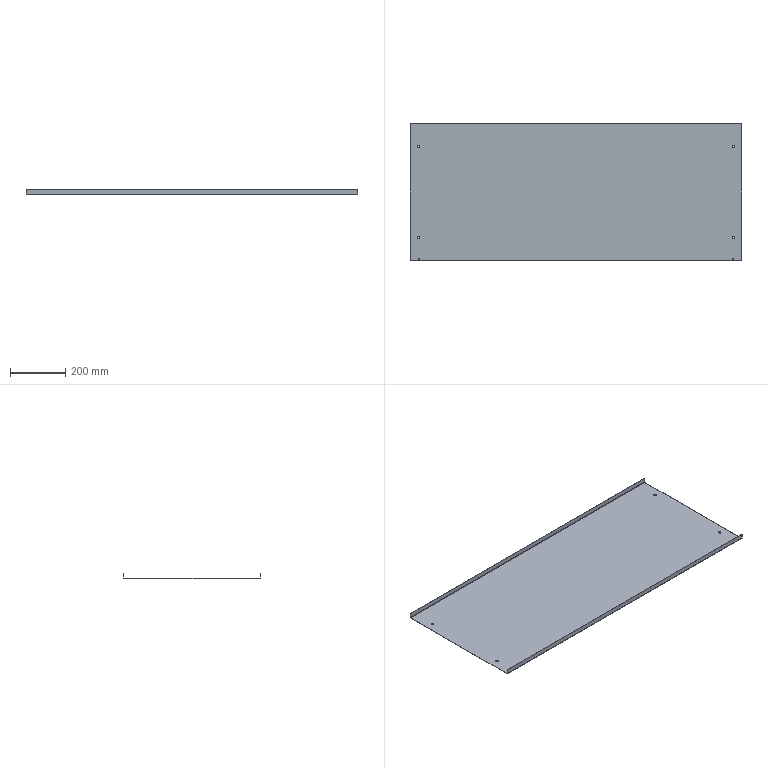Component | SolidWorks | TopPlate-1_TopPanelInnerPanel-2_TopPanelInnerPanel-1 | 1 solid | 34 faces | box 1198 x 498 x 18.5 mm | volume 509853 mm3 | plane 18 | cylinder 16 | commonest cylinder face diameters 8 x8 6 x4 2 x2 3.6 x2 | material 304
STEP:
#1=COLOUR_RGB('',0.7922,0.8196,0.9333);
#2=FILL_AREA_STYLE_COLOUR('',#1);
#3=FILL_AREA_STYLE('',(#2));
#4=SURFACE_STYLE_FILL_AREA(#3);
#5=SURFACE_SIDE_STYLE('',(#4));
#6=SURFACE_STYLE_USAGE(.BOTH.,#5);
#7=PRESENTATION_STYLE_ASSIGNMENT((#6));
#8=CARTESIAN_POINT('',(19.958,-8.263,78.498));
#9=VERTEX_POINT('',#8);
#10=CARTESIAN_POINT('',(19.958,-8.027,78.498));
#11=VERTEX_POINT('',#10);
#12=CARTESIAN_POINT('',(19.958,-8.145,78.498));
#13=DIRECTION('',(-0.,-0.,1.));
#14=DIRECTION('',(0.,1.,0.));
#15=AXIS2_PLACEMENT_3D('',#12,#13,#14);
#16=CIRCLE('',#15,0.1181);
#17=EDGE_CURVE('',#9,#11,#16,.T.);
#18=ORIENTED_EDGE('',*,*,#17,.T.);
#19=CARTESIAN_POINT('',(19.958,-8.027,78.467));
#20=VERTEX_POINT('',#19);
#21=CARTESIAN_POINT('',(19.958,-8.027,78.86));
#22=DIRECTION('',(0.,0.,-1.));
#23=VECTOR('',#22,39.37);
#24=LINE('',#21,#23);
#25=EDGE_CURVE('',#11,#20,#24,.T.);
#26=ORIENTED_EDGE('',*,*,#25,.T.);
#27=CARTESIAN_POINT('',(19.958,-8.263,78.467));
#28=VERTEX_POINT('',#27);
#29=CARTESIAN_POINT('',(19.958,-8.145,78.467));
#30=DIRECTION('',(0.,0.,-1.));
#31=DIRECTION('',(0.,-1.,0.));
#32=AXIS2_PLACEMENT_3D('',#29,#30,#31);
#33=CIRCLE('',#32,0.1181);
#34=EDGE_CURVE('',#20,#28,#33,.T.);
#35=ORIENTED_EDGE('',*,*,#34,.T.);
#36=CARTESIAN_POINT('',(19.958,-8.263,78.86));
#37=DIRECTION('',(0.,0.,-1.));
#38=VECTOR('',#37,39.37);
#39=LINE('',#36,#38);
#40=EDGE_CURVE('',#9,#28,#39,.T.);
#41=ORIENTED_EDGE('',*,*,#40,.F.);
#42=EDGE_LOOP('',(#18,#26,#35,#41));
#43=FACE_OUTER_BOUND('',#42,.T.);
#44=CARTESIAN_POINT('',(19.958,-8.145,78.86));
#45=DIRECTION('',(0.,0.,-1.));
#46=DIRECTION('',(0.,-1.,0.));
#47=AXIS2_PLACEMENT_3D('',#44,#45,#46);
#48=CYLINDRICAL_SURFACE('',#47,0.1181);
#49=ADVANCED_FACE('',(#43),#48,.F.);
#50=CARTESIAN_POINT('',(-24.688,-8.263,78.498));
#51=VERTEX_POINT('',#50);
#52=CARTESIAN_POINT('',(-24.688,-8.027,78.498));
#53=VERTEX_POINT('',#52);
#54=CARTESIAN_POINT('',(-24.688,-8.145,78.498));
#55=DIRECTION('',(-0.,-0.,1.));
#56=DIRECTION('',(0.,1.,0.));
#57=AXIS2_PLACEMENT_3D('',#54,#55,#56);
#58=CIRCLE('',#57,0.1181);
#59=EDGE_CURVE('',#51,#53,#58,.T.);
#60=ORIENTED_EDGE('',*,*,#59,.T.);
#61=CARTESIAN_POINT('',(-24.688,-8.027,78.467));
#62=VERTEX_POINT('',#61);
#63=CARTESIAN_POINT('',(-24.688,-8.027,78.86));
#64=DIRECTION('',(0.,0.,-1.));
#65=VECTOR('',#64,39.37);
#66=LINE('',#63,#65);
#67=EDGE_CURVE('',#53,#62,#66,.T.);
#68=ORIENTED_EDGE('',*,*,#67,.T.);
#69=CARTESIAN_POINT('',(-24.688,-8.263,78.467));
#70=VERTEX_POINT('',#69);
#71=CARTESIAN_POINT('',(-24.688,-8.145,78.467));
#72=DIRECTION('',(0.,0.,-1.));
#73=DIRECTION('',(0.,-1.,0.));
#74=AXIS2_PLACEMENT_3D('',#71,#72,#73);
#75=CIRCLE('',#74,0.1181);
#76=EDGE_CURVE('',#62,#70,#75,.T.);
#77=ORIENTED_EDGE('',*,*,#76,.T.);
#78=CARTESIAN_POINT('',(-24.688,-8.263,78.86));
#79=DIRECTION('',(0.,0.,-1.));
#80=VECTOR('',#79,39.37);
#81=LINE('',#78,#80);
#82=EDGE_CURVE('',#51,#70,#81,.T.);
#83=ORIENTED_EDGE('',*,*,#82,.F.);
#84=EDGE_LOOP('',(#60,#68,#77,#83));
#85=FACE_OUTER_BOUND('',#84,.T.);
#86=CARTESIAN_POINT('',(-24.688,-8.145,78.86));
#87=DIRECTION('',(0.,0.,-1.));
#88=DIRECTION('',(0.,-1.,0.));
#89=AXIS2_PLACEMENT_3D('',#86,#87,#88);
#90=CYLINDRICAL_SURFACE('',#89,0.1181);
#91=ADVANCED_FACE('',(#85),#90,.F.);
#92=CARTESIAN_POINT('',(-24.766,-5.29,78.498));
#93=VERTEX_POINT('',#92);
#94=CARTESIAN_POINT('',(-24.766,-4.975,78.498));
#95=VERTEX_POINT('',#94);
#96=CARTESIAN_POINT('',(-24.766,-5.133,78.498));
#97=DIRECTION('',(-0.,-0.,1.));
#98=DIRECTION('',(0.,1.,0.));
#99=AXIS2_PLACEMENT_3D('',#96,#97,#98);
#100=CIRCLE('',#99,0.1575);
#101=EDGE_CURVE('',#93,#95,#100,.T.);
#102=ORIENTED_EDGE('',*,*,#101,.T.);
#103=CARTESIAN_POINT('',(-24.766,-4.975,78.467));
#104=VERTEX_POINT('',#103);
#105=CARTESIAN_POINT('',(-24.766,-4.975,78.86));
#106=DIRECTION('',(0.,0.,-1.));
#107=VECTOR('',#106,39.37);
#108=LINE('',#105,#107);
#109=EDGE_CURVE('',#95,#104,#108,.T.);
#110=ORIENTED_EDGE('',*,*,#109,.T.);
#111=CARTESIAN_POINT('',(-24.766,-5.29,78.467));
#112=VERTEX_POINT('',#111);
#113=CARTESIAN_POINT('',(-24.766,-5.133,78.467));
#114=DIRECTION('',(0.,0.,-1.));
#115=DIRECTION('',(0.,1.,0.));
#116=AXIS2_PLACEMENT_3D('',#113,#114,#115);
#117=CIRCLE('',#116,0.1575);
#118=EDGE_CURVE('',#104,#112,#117,.T.);
#119=ORIENTED_EDGE('',*,*,#118,.T.);
#120=CARTESIAN_POINT('',(-24.766,-5.29,78.86));
#121=DIRECTION('',(0.,0.,-1.));
#122=VECTOR('',#121,39.37);
#123=LINE('',#120,#122);
#124=EDGE_CURVE('',#93,#112,#123,.T.);
#125=ORIENTED_EDGE('',*,*,#124,.F.);
#126=EDGE_LOOP('',(#102,#110,#119,#125));
#127=FACE_OUTER_BOUND('',#126,.T.);
#128=CARTESIAN_POINT('',(-24.766,-5.133,78.86));
#129=DIRECTION('',(0.,0.,-1.));
#130=DIRECTION('',(0.,-1.,0.));
#131=AXIS2_PLACEMENT_3D('',#128,#129,#130);
#132=CYLINDRICAL_SURFACE('',#131,0.1575);
#133=ADVANCED_FACE('',(#127),#132,.F.);
#134=CARTESIAN_POINT('',(-24.766,7.702,78.498));
#135=VERTEX_POINT('',#134);
#136=CARTESIAN_POINT('',(-24.766,8.017,78.498));
#137=VERTEX_POINT('',#136);
#138=CARTESIAN_POINT('',(-24.766,7.859,78.498));
#139=DIRECTION('',(-0.,-0.,1.));
#140=DIRECTION('',(0.,1.,0.));
#141=AXIS2_PLACEMENT_3D('',#138,#139,#140);
#142=CIRCLE('',#141,0.1575);
#143=EDGE_CURVE('',#135,#137,#142,.T.);
#144=ORIENTED_EDGE('',*,*,#143,.T.);
#145=CARTESIAN_POINT('',(-24.766,8.017,78.467));
#146=VERTEX_POINT('',#145);
#147=CARTESIAN_POINT('',(-24.766,8.017,78.86));
#148=DIRECTION('',(0.,0.,-1.));
#149=VECTOR('',#148,39.37);
#150=LINE('',#147,#149);
#151=EDGE_CURVE('',#137,#146,#150,.T.);
#152=ORIENTED_EDGE('',*,*,#151,.T.);
#153=CARTESIAN_POINT('',(-24.766,7.702,78.467));
#154=VERTEX_POINT('',#153);
#155=CARTESIAN_POINT('',(-24.766,7.859,78.467));
#156=DIRECTION('',(0.,0.,-1.));
#157=DIRECTION('',(0.,1.,0.));
#158=AXIS2_PLACEMENT_3D('',#155,#156,#157);
#159=CIRCLE('',#158,0.1575);
#160=EDGE_CURVE('',#146,#154,#159,.T.);
#161=ORIENTED_EDGE('',*,*,#160,.T.);
#162=CARTESIAN_POINT('',(-24.766,7.702,78.86));
#163=DIRECTION('',(0.,0.,-1.));
#164=VECTOR('',#163,39.37);
#165=LINE('',#162,#164);
#166=EDGE_CURVE('',#135,#154,#165,.T.);
#167=ORIENTED_EDGE('',*,*,#166,.F.);
#168=EDGE_LOOP('',(#144,#152,#161,#167));
#169=FACE_OUTER_BOUND('',#168,.T.);
#170=CARTESIAN_POINT('',(-24.766,7.859,78.86));
#171=DIRECTION('',(0.,0.,-1.));
#172=DIRECTION('',(0.,-1.,0.));
#173=AXIS2_PLACEMENT_3D('',#170,#171,#172);
#174=CYLINDRICAL_SURFACE('',#173,0.1575);
#175=ADVANCED_FACE('',(#169),#174,.F.);
#176=CARTESIAN_POINT('',(20.037,7.702,78.498));
#177=VERTEX_POINT('',#176);
#178=CARTESIAN_POINT('',(20.037,8.017,78.498));
#179=VERTEX_POINT('',#178);
#180=CARTESIAN_POINT('',(20.037,7.859,78.498));
#181=DIRECTION('',(-0.,-0.,1.));
#182=DIRECTION('',(0.,1.,0.));
#183=AXIS2_PLACEMENT_3D('',#180,#181,#182);
#184=CIRCLE('',#183,0.1575);
#185=EDGE_CURVE('',#177,#179,#184,.T.);
#186=ORIENTED_EDGE('',*,*,#185,.T.);
#187=CARTESIAN_POINT('',(20.037,8.017,78.467));
#188=VERTEX_POINT('',#187);
#189=CARTESIAN_POINT('',(20.037,8.017,78.86));
#190=DIRECTION('',(0.,0.,-1.));
#191=VECTOR('',#190,39.37);
#192=LINE('',#189,#191);
#193=EDGE_CURVE('',#179,#188,#192,.T.);
#194=ORIENTED_EDGE('',*,*,#193,.T.);
#195=CARTESIAN_POINT('',(20.037,7.702,78.467));
#196=VERTEX_POINT('',#195);
#197=CARTESIAN_POINT('',(20.037,7.859,78.467));
#198=DIRECTION('',(0.,0.,-1.));
#199=DIRECTION('',(0.,-1.,0.));
#200=AXIS2_PLACEMENT_3D('',#197,#198,#199);
#201=CIRCLE('',#200,0.1575);
#202=EDGE_CURVE('',#188,#196,#201,.T.);
#203=ORIENTED_EDGE('',*,*,#202,.T.);
#204=CARTESIAN_POINT('',(20.037,7.702,78.86));
#205=DIRECTION('',(0.,0.,-1.));
#206=VECTOR('',#205,39.37);
#207=LINE('',#204,#206);
#208=EDGE_CURVE('',#177,#196,#207,.T.);
#209=ORIENTED_EDGE('',*,*,#208,.F.);
#210=EDGE_LOOP('',(#186,#194,#203,#209));
#211=FACE_OUTER_BOUND('',#210,.T.);
#212=CARTESIAN_POINT('',(20.037,7.859,78.86));
#213=DIRECTION('',(0.,0.,-1.));
#214=DIRECTION('',(0.,-1.,0.));
#215=AXIS2_PLACEMENT_3D('',#212,#213,#214);
#216=CYLINDRICAL_SURFACE('',#215,0.1575);
#217=ADVANCED_FACE('',(#211),#216,.F.);
#218=CARTESIAN_POINT('',(20.037,-5.29,78.498));
#219=VERTEX_POINT('',#218);
#220=CARTESIAN_POINT('',(20.037,-4.975,78.498));
#221=VERTEX_POINT('',#220);
#222=CARTESIAN_POINT('',(20.037,-5.133,78.498));
#223=DIRECTION('',(-0.,-0.,1.));
#224=DIRECTION('',(0.,1.,0.));
#225=AXIS2_PLACEMENT_3D('',#222,#223,#224);
#226=CIRCLE('',#225,0.1575);
#227=EDGE_CURVE('',#219,#221,#226,.T.);
#228=ORIENTED_EDGE('',*,*,#227,.T.);
#229=CARTESIAN_POINT('',(20.037,-4.975,78.467));
#230=VERTEX_POINT('',#229);
#231=CARTESIAN_POINT('',(20.037,-4.975,78.86));
#232=DIRECTION('',(0.,0.,-1.));
#233=VECTOR('',#232,39.37);
#234=LINE('',#231,#233);
#235=EDGE_CURVE('',#221,#230,#234,.T.);
#236=ORIENTED_EDGE('',*,*,#235,.T.);
#237=CARTESIAN_POINT('',(20.037,-5.29,78.467));
#238=VERTEX_POINT('',#237);
#239=CARTESIAN_POINT('',(20.037,-5.133,78.467));
#240=DIRECTION('',(0.,0.,-1.));
#241=DIRECTION('',(0.,-1.,0.));
#242=AXIS2_PLACEMENT_3D('',#239,#240,#241);
#243=CIRCLE('',#242,0.1575);
#244=EDGE_CURVE('',#230,#238,#243,.T.);
#245=ORIENTED_EDGE('',*,*,#244,.T.);
#246=CARTESIAN_POINT('',(20.037,-5.29,78.86));
#247=DIRECTION('',(0.,0.,-1.));
#248=VECTOR('',#247,39.37);
#249=LINE('',#246,#248);
#250=EDGE_CURVE('',#219,#238,#249,.T.);
#251=ORIENTED_EDGE('',*,*,#250,.F.);
#252=EDGE_LOOP('',(#228,#236,#245,#251));
#253=FACE_OUTER_BOUND('',#252,.T.);
#254=CARTESIAN_POINT('',(20.037,-5.133,78.86));
#255=DIRECTION('',(0.,0.,-1.));
#256=DIRECTION('',(0.,-1.,0.));
#257=AXIS2_PLACEMENT_3D('',#254,#255,#256);
#258=CYLINDRICAL_SURFACE('',#257,0.1575);
#259=ADVANCED_FACE('',(#253),#258,.F.);
#260=CARTESIAN_POINT('',(-25.948,-8.369,78.467));
#261=VERTEX_POINT('',#260);
#262=CARTESIAN_POINT('',(-25.948,-8.369,78.498));
#263=VERTEX_POINT('',#262);
#264=CARTESIAN_POINT('',(-25.948,-8.369,78.467));
#265=DIRECTION('',(-0.,-0.,1.));
#266=VECTOR('',#265,39.37);
#267=LINE('',#264,#266);
#268=EDGE_CURVE('',#261,#263,#267,.T.);
#269=ORIENTED_EDGE('',*,*,#268,.F.);
#270=CARTESIAN_POINT('',(-25.948,-8.44,78.537));
#271=VERTEX_POINT('',#270);
#272=CARTESIAN_POINT('',(-25.948,-8.369,78.537));
#273=DIRECTION('',(-1.,0.,-0.));
#274=DIRECTION('',(0.,0.,1.));
#275=AXIS2_PLACEMENT_3D('',#272,#273,#274);
#276=CIRCLE('',#275,0.07087);
#277=EDGE_CURVE('',#261,#271,#276,.T.);
#278=ORIENTED_EDGE('',*,*,#277,.T.);
#279=CARTESIAN_POINT('',(-25.948,-8.408,78.537));
#280=VERTEX_POINT('',#279);
#281=CARTESIAN_POINT('',(-25.948,-8.408,78.537));
#282=DIRECTION('',(-0.,-1.,-0.));
#283=VECTOR('',#282,39.37);
#284=LINE('',#281,#283);
#285=EDGE_CURVE('',#280,#271,#284,.T.);
#286=ORIENTED_EDGE('',*,*,#285,.F.);
#287=CARTESIAN_POINT('',(-25.948,-8.369,78.537));
#288=DIRECTION('',(-1.,0.,-0.));
#289=DIRECTION('',(0.,1.,0.));
#290=AXIS2_PLACEMENT_3D('',#287,#288,#289);
#291=CIRCLE('',#290,0.03937);
#292=EDGE_CURVE('',#263,#280,#291,.T.);
#293=ORIENTED_EDGE('',*,*,#292,.F.);
#294=EDGE_LOOP('',(#269,#278,#286,#293));
#295=FACE_OUTER_BOUND('',#294,.T.);
#296=CARTESIAN_POINT('',(-25.948,-8.369,78.467));
#297=DIRECTION('',(-1.,0.,-0.));
#298=DIRECTION('',(-0.,-0.,1.));
#299=AXIS2_PLACEMENT_3D('',#296,#297,#298);
#300=PLANE('',#299);
#301=ADVANCED_FACE('',(#295),#300,.T.);
#302=CARTESIAN_POINT('',(-25.948,11.095,78.467));
#303=VERTEX_POINT('',#302);
#304=CARTESIAN_POINT('',(-25.948,-8.44,78.467));
#305=DIRECTION('',(-0.,-1.,-0.));
#306=VECTOR('',#305,39.37);
#307=LINE('',#304,#306);
#308=EDGE_CURVE('',#303,#261,#307,.T.);
#309=ORIENTED_EDGE('',*,*,#308,.T.);
#310=ORIENTED_EDGE('',*,*,#268,.T.);
#311=CARTESIAN_POINT('',(-25.948,11.095,78.498));
#312=VERTEX_POINT('',#311);
#313=CARTESIAN_POINT('',(-25.948,-8.44,78.498));
#314=DIRECTION('',(-0.,-1.,-0.));
#315=VECTOR('',#314,39.37);
#316=LINE('',#313,#315);
#317=EDGE_CURVE('',#312,#263,#316,.T.);
#318=ORIENTED_EDGE('',*,*,#317,.F.);
#319=CARTESIAN_POINT('',(-25.948,11.095,78.498));
#320=DIRECTION('',(0.,0.,-1.));
#321=VECTOR('',#320,39.37);
#322=LINE('',#319,#321);
#323=EDGE_CURVE('',#312,#303,#322,.T.);
#324=ORIENTED_EDGE('',*,*,#323,.T.);
#325=EDGE_LOOP('',(#309,#310,#318,#324));
#326=FACE_OUTER_BOUND('',#325,.T.);
#327=CARTESIAN_POINT('',(-25.948,-8.408,78.537));
#328=DIRECTION('',(-1.,0.,-0.));
#329=DIRECTION('',(-0.,-0.,1.));
#330=AXIS2_PLACEMENT_3D('',#327,#328,#329);
#331=PLANE('',#330);
#332=ADVANCED_FACE('',(#326),#331,.T.);
#333=CARTESIAN_POINT('',(21.218,-8.44,78.537));
#334=VERTEX_POINT('',#333);
#335=CARTESIAN_POINT('',(21.218,-8.408,78.537));
#336=VERTEX_POINT('',#335);
#337=CARTESIAN_POINT('',(21.218,-8.44,78.537));
#338=DIRECTION('',(0.,1.,0.));
#339=VECTOR('',#338,39.37);
#340=LINE('',#337,#339);
#341=EDGE_CURVE('',#334,#336,#340,.T.);
#342=ORIENTED_EDGE('',*,*,#341,.F.);
#343=CARTESIAN_POINT('',(21.218,-8.369,78.467));
#344=VERTEX_POINT('',#343);
#345=CARTESIAN_POINT('',(21.218,-8.369,78.537));
#346=DIRECTION('',(-1.,0.,-0.));
#347=DIRECTION('',(0.,0.,1.));
#348=AXIS2_PLACEMENT_3D('',#345,#346,#347);
#349=CIRCLE('',#348,0.07087);
#350=EDGE_CURVE('',#344,#334,#349,.T.);
#351=ORIENTED_EDGE('',*,*,#350,.F.);
#352=CARTESIAN_POINT('',(21.218,-8.369,78.498));
#353=VERTEX_POINT('',#352);
#354=CARTESIAN_POINT('',(21.218,-8.369,78.498));
#355=DIRECTION('',(0.,0.,-1.));
#356=VECTOR('',#355,39.37);
#357=LINE('',#354,#356);
#358=EDGE_CURVE('',#353,#344,#357,.T.);
#359=ORIENTED_EDGE('',*,*,#358,.F.);
#360=CARTESIAN_POINT('',(21.218,-8.369,78.537));
#361=DIRECTION('',(-1.,0.,-0.));
#362=DIRECTION('',(0.,1.,0.));
#363=AXIS2_PLACEMENT_3D('',#360,#361,#362);
#364=CIRCLE('',#363,0.03937);
#365=EDGE_CURVE('',#353,#336,#364,.T.);
#366=ORIENTED_EDGE('',*,*,#365,.T.);
#367=EDGE_LOOP('',(#342,#351,#359,#366));
#368=FACE_OUTER_BOUND('',#367,.T.);
#369=CARTESIAN_POINT('',(21.218,-8.44,78.537));
#370=DIRECTION('',(1.,-0.,0.));
#371=DIRECTION('',(0.,0.,-1.));
#372=AXIS2_PLACEMENT_3D('',#369,#370,#371);
#373=PLANE('',#372);
#374=ADVANCED_FACE('',(#368),#373,.T.);
#375=CARTESIAN_POINT('',(21.218,-8.44,79.195));
#376=VERTEX_POINT('',#375);
#377=CARTESIAN_POINT('',(21.218,-8.44,79.195));
#378=DIRECTION('',(-0.,-0.,1.));
#379=VECTOR('',#378,39.37);
#380=LINE('',#377,#379);
#381=EDGE_CURVE('',#334,#376,#380,.T.);
#382=ORIENTED_EDGE('',*,*,#381,.F.);
#383=ORIENTED_EDGE('',*,*,#341,.T.);
#384=CARTESIAN_POINT('',(21.218,-8.408,79.195));
#385=VERTEX_POINT('',#384);
#386=CARTESIAN_POINT('',(21.218,-8.408,79.195));
#387=DIRECTION('',(-0.,-0.,1.));
#388=VECTOR('',#387,39.37);
#389=LINE('',#386,#388);
#390=EDGE_CURVE('',#336,#385,#389,.T.);
#391=ORIENTED_EDGE('',*,*,#390,.T.);
#392=CARTESIAN_POINT('',(21.218,-8.408,79.195));
#393=DIRECTION('',(-0.,-1.,-0.));
#394=VECTOR('',#393,39.37);
#395=LINE('',#392,#394);
#396=EDGE_CURVE('',#385,#376,#395,.T.);
#397=ORIENTED_EDGE('',*,*,#396,.T.);
#398=EDGE_LOOP('',(#382,#383,#391,#397));
#399=FACE_OUTER_BOUND('',#398,.T.);
#400=CARTESIAN_POINT('',(21.218,-8.369,78.498));
#401=DIRECTION('',(1.,-0.,0.));
#402=DIRECTION('',(0.,0.,-1.));
#403=AXIS2_PLACEMENT_3D('',#400,#401,#402);
#404=PLANE('',#403);
#405=ADVANCED_FACE('',(#399),#404,.T.);
#406=CARTESIAN_POINT('',(-25.948,11.166,78.537));
#407=VERTEX_POINT('',#406);
#408=CARTESIAN_POINT('',(-25.948,11.135,78.537));
#409=VERTEX_POINT('',#408);
#410=CARTESIAN_POINT('',(-25.948,11.166,78.537));
#411=DIRECTION('',(-0.,-1.,-0.));
#412=VECTOR('',#411,39.37);
#413=LINE('',#410,#412);
#414=EDGE_CURVE('',#407,#409,#413,.T.);
#415=ORIENTED_EDGE('',*,*,#414,.F.);
#416=CARTESIAN_POINT('',(-25.948,11.095,78.537));
#417=DIRECTION('',(-1.,0.,-0.));
#418=DIRECTION('',(0.,0.,1.));
#419=AXIS2_PLACEMENT_3D('',#416,#417,#418);
#420=CIRCLE('',#419,0.07087);
#421=EDGE_CURVE('',#407,#303,#420,.T.);
#422=ORIENTED_EDGE('',*,*,#421,.T.);
#423=ORIENTED_EDGE('',*,*,#323,.F.);
#424=CARTESIAN_POINT('',(-25.948,11.095,78.537));
#425=DIRECTION('',(-1.,0.,-0.));
#426=DIRECTION('',(0.,1.,0.));
#427=AXIS2_PLACEMENT_3D('',#424,#425,#426);
#428=CIRCLE('',#427,0.03937);
#429=EDGE_CURVE('',#409,#312,#428,.T.);
#430=ORIENTED_EDGE('',*,*,#429,.F.);
#431=EDGE_LOOP('',(#415,#422,#423,#430));
#432=FACE_OUTER_BOUND('',#431,.T.);
#433=CARTESIAN_POINT('',(-25.948,11.166,78.537));
#434=DIRECTION('',(-1.,0.,-0.));
#435=DIRECTION('',(-0.,-0.,1.));
#436=AXIS2_PLACEMENT_3D('',#433,#434,#435);
#437=PLANE('',#436);
#438=ADVANCED_FACE('',(#432),#437,.T.);
#439=CARTESIAN_POINT('',(-25.948,11.166,79.195));
#440=VERTEX_POINT('',#439);
#441=CARTESIAN_POINT('',(-25.948,11.166,79.195));
#442=DIRECTION('',(0.,0.,-1.));
#443=VECTOR('',#442,39.37);
#444=LINE('',#441,#443);
#445=EDGE_CURVE('',#440,#407,#444,.T.);
#446=ORIENTED_EDGE('',*,*,#445,.T.);
#447=ORIENTED_EDGE('',*,*,#414,.T.);
#448=CARTESIAN_POINT('',(-25.948,11.135,79.195));
#449=VERTEX_POINT('',#448);
#450=CARTESIAN_POINT('',(-25.948,11.135,79.195));
#451=DIRECTION('',(0.,0.,-1.));
#452=VECTOR('',#451,39.37);
#453=LINE('',#450,#452);
#454=EDGE_CURVE('',#449,#409,#453,.T.);
#455=ORIENTED_EDGE('',*,*,#454,.F.);
#456=CARTESIAN_POINT('',(-25.948,11.166,79.195));
#457=DIRECTION('',(-0.,-1.,-0.));
#458=VECTOR('',#457,39.37);
#459=LINE('',#456,#458);
#460=EDGE_CURVE('',#440,#449,#459,.T.);
#461=ORIENTED_EDGE('',*,*,#460,.F.);
#462=EDGE_LOOP('',(#446,#447,#455,#461));
#463=FACE_OUTER_BOUND('',#462,.T.);
#464=CARTESIAN_POINT('',(-25.948,11.095,78.498));
#465=DIRECTION('',(-1.,0.,-0.));
#466=DIRECTION('',(-0.,-0.,1.));
#467=AXIS2_PLACEMENT_3D('',#464,#465,#466);
#468=PLANE('',#467);
#469=ADVANCED_FACE('',(#463),#468,.T.);
#470=CARTESIAN_POINT('',(21.218,11.095,78.467));
#471=VERTEX_POINT('',#470);
#472=CARTESIAN_POINT('',(21.218,11.095,78.498));
#473=VERTEX_POINT('',#472);
#474=CARTESIAN_POINT('',(21.218,11.095,78.467));
#475=DIRECTION('',(-0.,-0.,1.));
#476=VECTOR('',#475,39.37);
#477=LINE('',#474,#476);
#478=EDGE_CURVE('',#471,#473,#477,.T.);
#479=ORIENTED_EDGE('',*,*,#478,.F.);
#480=CARTESIAN_POINT('',(21.218,11.166,78.537));
#481=VERTEX_POINT('',#480);
#482=CARTESIAN_POINT('',(21.218,11.095,78.537));
#483=DIRECTION('',(-1.,0.,-0.));
#484=DIRECTION('',(0.,0.,1.));
#485=AXIS2_PLACEMENT_3D('',#482,#483,#484);
#486=CIRCLE('',#485,0.07087);
#487=EDGE_CURVE('',#481,#471,#486,.T.);
#488=ORIENTED_EDGE('',*,*,#487,.F.);
#489=CARTESIAN_POINT('',(21.218,11.135,78.537));
#490=VERTEX_POINT('',#489);
#491=CARTESIAN_POINT('',(21.218,11.135,78.537));
#492=DIRECTION('',(0.,1.,0.));
#493=VECTOR('',#492,39.37);
#494=LINE('',#491,#493);
#495=EDGE_CURVE('',#490,#481,#494,.T.);
#496=ORIENTED_EDGE('',*,*,#495,.F.);
#497=CARTESIAN_POINT('',(21.218,11.095,78.537));
#498=DIRECTION('',(-1.,0.,-0.));
#499=DIRECTION('',(0.,1.,0.));
#500=AXIS2_PLACEMENT_3D('',#497,#498,#499);
#501=CIRCLE('',#500,0.03937);
#502=EDGE_CURVE('',#490,#473,#501,.T.);
#503=ORIENTED_EDGE('',*,*,#502,.T.);
#504=EDGE_LOOP('',(#479,#488,#496,#503));
#505=FACE_OUTER_BOUND('',#504,.T.);
#506=CARTESIAN_POINT('',(21.218,11.095,78.467));
#507=DIRECTION('',(1.,-0.,0.));
#508=DIRECTION('',(0.,0.,-1.));
#509=AXIS2_PLACEMENT_3D('',#506,#507,#508);
#510=PLANE('',#509);
#511=ADVANCED_FACE('',(#505),#510,.T.);
#512=CARTESIAN_POINT('',(21.218,-8.44,78.467));
#513=DIRECTION('',(-0.,-1.,-0.));
#514=VECTOR('',#513,39.37);
#515=LINE('',#512,#514);
#516=EDGE_CURVE('',#471,#344,#515,.T.);
#517=ORIENTED_EDGE('',*,*,#516,.F.);
#518=ORIENTED_EDGE('',*,*,#478,.T.);
#519=CARTESIAN_POINT('',(21.218,-8.44,78.498));
#520=DIRECTION('',(-0.,-1.,-0.));
#521=VECTOR('',#520,39.37);
#522=LINE('',#519,#521);
#523=EDGE_CURVE('',#473,#353,#522,.T.);
#524=ORIENTED_EDGE('',*,*,#523,.T.);
#525=ORIENTED_EDGE('',*,*,#358,.T.);
#526=EDGE_LOOP('',(#517,#518,#524,#525));
#527=FACE_OUTER_BOUND('',#526,.T.);
#528=CARTESIAN_POINT('',(21.218,11.135,78.537));
#529=DIRECTION('',(1.,-0.,0.));
#530=DIRECTION('',(0.,0.,-1.));
#531=AXIS2_PLACEMENT_3D('',#528,#529,#530);
#532=PLANE('',#531);
#533=ADVANCED_FACE('',(#527),#532,.T.);
#534=ORIENTED_EDGE('',*,*,#381,.T.);
#535=CARTESIAN_POINT('',(-25.948,-8.44,79.195));
#536=VERTEX_POINT('',#535);
#537=CARTESIAN_POINT('',(-25.948,-8.44,79.195));
#538=DIRECTION('',(1.,-0.,0.));
#539=VECTOR('',#538,39.37);
#540=LINE('',#537,#539);
#541=EDGE_CURVE('',#536,#376,#540,.T.);
#542=ORIENTED_EDGE('',*,*,#541,.F.);
#543=CARTESIAN_POINT('',(-25.948,-8.44,79.195));
#544=DIRECTION('',(-0.,-0.,1.));
#545=VECTOR('',#544,39.37);
#546=LINE('',#543,#545);
#547=EDGE_CURVE('',#271,#536,#546,.T.);
#548=ORIENTED_EDGE('',*,*,#547,.F.);
#549=CARTESIAN_POINT('',(-25.948,-8.44,78.537));
#550=DIRECTION('',(1.,-0.,0.));
#551=VECTOR('',#550,39.37);
#552=LINE('',#549,#551);
#553=EDGE_CURVE('',#271,#334,#552,.T.);
#554=ORIENTED_EDGE('',*,*,#553,.T.);
#555=EDGE_LOOP('',(#534,#542,#548,#554));
#556=FACE_OUTER_BOUND('',#555,.T.);
#557=CARTESIAN_POINT('',(-25.948,-8.44,79.195));
#558=DIRECTION('',(0.,1.,0.));
#559=DIRECTION('',(0.,0.,-1.));
#560=AXIS2_PLACEMENT_3D('',#557,#558,#559);
#561=PLANE('',#560);
#562=ADVANCED_FACE('',(#556),#561,.F.);
#563=ORIENTED_EDGE('',*,*,#396,.F.);
#564=CARTESIAN_POINT('',(-25.948,-8.408,79.195));
#565=VERTEX_POINT('',#564);
#566=CARTESIAN_POINT('',(-25.948,-8.408,79.195));
#567=DIRECTION('',(1.,-0.,0.));
#568=VECTOR('',#567,39.37);
#569=LINE('',#566,#568);
#570=EDGE_CURVE('',#565,#385,#569,.T.);
#571=ORIENTED_EDGE('',*,*,#570,.F.);
#572=CARTESIAN_POINT('',(-25.948,-8.408,79.195));
#573=DIRECTION('',(-0.,-1.,-0.));
#574=VECTOR('',#573,39.37);
#575=LINE('',#572,#574);
#576=EDGE_CURVE('',#565,#536,#575,.T.);
#577=ORIENTED_EDGE('',*,*,#576,.T.);
#578=ORIENTED_EDGE('',*,*,#541,.T.);
#579=EDGE_LOOP('',(#563,#571,#577,#578));
#580=FACE_OUTER_BOUND('',#579,.T.);
#581=CARTESIAN_POINT('',(-25.948,-8.408,79.195));
#582=DIRECTION('',(-0.,-0.,1.));
#583=DIRECTION('',(0.,1.,0.));
#584=AXIS2_PLACEMENT_3D('',#581,#582,#583);
#585=PLANE('',#584);
#586=ADVANCED_FACE('',(#580),#585,.T.);
#587=ORIENTED_EDGE('',*,*,#390,.F.);
#588=CARTESIAN_POINT('',(-25.948,-8.408,78.537));
#589=DIRECTION('',(1.,-0.,0.));
#590=VECTOR('',#589,39.37);
#591=LINE('',#588,#590);
#592=EDGE_CURVE('',#280,#336,#591,.T.);
#593=ORIENTED_EDGE('',*,*,#592,.F.);
#594=CARTESIAN_POINT('',(-25.948,-8.408,79.195));
#595=DIRECTION('',(-0.,-0.,1.));
#596=VECTOR('',#595,39.37);
#597=LINE('',#594,#596);
#598=EDGE_CURVE('',#280,#565,#597,.T.);
#599=ORIENTED_EDGE('',*,*,#598,.T.);
#600=ORIENTED_EDGE('',*,*,#570,.T.);
#601=EDGE_LOOP('',(#587,#593,#599,#600));
#602=FACE_OUTER_BOUND('',#601,.T.);
#603=CARTESIAN_POINT('',(-25.948,-8.408,79.195));
#604=DIRECTION('',(0.,1.,0.));
#605=DIRECTION('',(0.,0.,-1.));
#606=AXIS2_PLACEMENT_3D('',#603,#604,#605);
#607=PLANE('',#606);
#608=ADVANCED_FACE('',(#602),#607,.T.);
#609=ORIENTED_EDGE('',*,*,#365,.F.);
#610=CARTESIAN_POINT('',(-25.948,-8.369,78.498));
#611=DIRECTION('',(1.,-0.,0.));
#612=VECTOR('',#611,39.37);
#613=LINE('',#610,#612);
#614=EDGE_CURVE('',#263,#353,#613,.T.);
#615=ORIENTED_EDGE('',*,*,#614,.F.);
#616=ORIENTED_EDGE('',*,*,#292,.T.);
#617=ORIENTED_EDGE('',*,*,#592,.T.);
#618=EDGE_LOOP('',(#609,#615,#616,#617));
#619=FACE_OUTER_BOUND('',#618,.T.);
#620=CARTESIAN_POINT('',(-25.948,-8.369,78.537));
#621=DIRECTION('',(1.,-0.,0.));
#622=DIRECTION('',(0.,0.,-1.));
#623=AXIS2_PLACEMENT_3D('',#620,#621,#622);
#624=CYLINDRICAL_SURFACE('',#623,0.03937);
#625=ADVANCED_FACE('',(#619),#624,.F.);
#626=ORIENTED_EDGE('',*,*,#17,.F.);
#627=CARTESIAN_POINT('',(19.958,-8.145,78.498));
#628=DIRECTION('',(-0.,-0.,1.));
#629=DIRECTION('',(0.,1.,0.));
#630=AXIS2_PLACEMENT_3D('',#627,#628,#629);
#631=CIRCLE('',#630,0.1181);
#632=EDGE_CURVE('',#11,#9,#631,.T.);
#633=ORIENTED_EDGE('',*,*,#632,.F.);
#634=EDGE_LOOP('',(#626,#633));
#635=FACE_BOUND('',#634,.T.);
#636=ORIENTED_EDGE('',*,*,#59,.F.);
#637=CARTESIAN_POINT('',(-24.688,-8.145,78.498));
#638=DIRECTION('',(-0.,-0.,1.));
#639=DIRECTION('',(0.,1.,0.));
#640=AXIS2_PLACEMENT_3D('',#637,#638,#639);
#641=CIRCLE('',#640,0.1181);
#642=EDGE_CURVE('',#53,#51,#641,.T.);
#643=ORIENTED_EDGE('',*,*,#642,.F.);
#644=EDGE_LOOP('',(#636,#643));
#645=FACE_BOUND('',#644,.T.);
#646=ORIENTED_EDGE('',*,*,#101,.F.);
#647=CARTESIAN_POINT('',(-24.766,-5.133,78.498));
#648=DIRECTION('',(-0.,-0.,1.));
#649=DIRECTION('',(0.,1.,0.));
#650=AXIS2_PLACEMENT_3D('',#647,#648,#649);
#651=CIRCLE('',#650,0.1575);
#652=EDGE_CURVE('',#95,#93,#651,.T.);
#653=ORIENTED_EDGE('',*,*,#652,.F.);
#654=EDGE_LOOP('',(#646,#653));
#655=FACE_BOUND('',#654,.T.);
#656=ORIENTED_EDGE('',*,*,#143,.F.);
#657=CARTESIAN_POINT('',(-24.766,7.859,78.498));
#658=DIRECTION('',(-0.,-0.,1.));
#659=DIRECTION('',(0.,1.,0.));
#660=AXIS2_PLACEMENT_3D('',#657,#658,#659);
#661=CIRCLE('',#660,0.1575);
#662=EDGE_CURVE('',#137,#135,#661,.T.);
#663=ORIENTED_EDGE('',*,*,#662,.F.);
#664=EDGE_LOOP('',(#656,#663));
#665=FACE_BOUND('',#664,.T.);
#666=ORIENTED_EDGE('',*,*,#185,.F.);
#667=CARTESIAN_POINT('',(20.037,7.859,78.498));
#668=DIRECTION('',(-0.,-0.,1.));
#669=DIRECTION('',(0.,1.,0.));
#670=AXIS2_PLACEMENT_3D('',#667,#668,#669);
#671=CIRCLE('',#670,0.1575);
#672=EDGE_CURVE('',#179,#177,#671,.T.);
#673=ORIENTED_EDGE('',*,*,#672,.F.);
#674=EDGE_LOOP('',(#666,#673));
#675=FACE_BOUND('',#674,.T.);
#676=ORIENTED_EDGE('',*,*,#227,.F.);
#677=CARTESIAN_POINT('',(20.037,-5.133,78.498));
#678=DIRECTION('',(-0.,-0.,1.));
#679=DIRECTION('',(0.,1.,0.));
#680=AXIS2_PLACEMENT_3D('',#677,#678,#679);
#681=CIRCLE('',#680,0.1575);
#682=EDGE_CURVE('',#221,#219,#681,.T.);
#683=ORIENTED_EDGE('',*,*,#682,.F.);
#684=EDGE_LOOP('',(#676,#683));
#685=FACE_BOUND('',#684,.T.);
#686=ORIENTED_EDGE('',*,*,#523,.F.);
#687=CARTESIAN_POINT('',(-25.948,11.095,78.498));
#688=DIRECTION('',(1.,-0.,0.));
#689=VECTOR('',#688,39.37);
#690=LINE('',#687,#689);
#691=EDGE_CURVE('',#312,#473,#690,.T.);
#692=ORIENTED_EDGE('',*,*,#691,.F.);
#693=ORIENTED_EDGE('',*,*,#317,.T.);
#694=ORIENTED_EDGE('',*,*,#614,.T.);
#695=EDGE_LOOP('',(#686,#692,#693,#694));
#696=FACE_OUTER_BOUND('',#695,.T.);
#697=CARTESIAN_POINT('',(-25.948,-8.44,78.498));
#698=DIRECTION('',(-0.,-0.,1.));
#699=DIRECTION('',(0.,1.,0.));
#700=AXIS2_PLACEMENT_3D('',#697,#698,#699);
#701=PLANE('',#700);
#702=ADVANCED_FACE('',(#635,#645,#655,#665,#675,#685,#696),#701,.T.);
#703=ORIENTED_EDGE('',*,*,#502,.F.);
#704=CARTESIAN_POINT('',(-25.948,11.135,78.537));
#705=DIRECTION('',(1.,-0.,0.));
#706=VECTOR('',#705,39.37);
#707=LINE('',#704,#706);
#708=EDGE_CURVE('',#409,#490,#707,.T.);
#709=ORIENTED_EDGE('',*,*,#708,.F.);
#710=ORIENTED_EDGE('',*,*,#429,.T.);
#711=ORIENTED_EDGE('',*,*,#691,.T.);
#712=EDGE_LOOP('',(#703,#709,#710,#711));
#713=FACE_OUTER_BOUND('',#712,.T.);
#714=CARTESIAN_POINT('',(-25.948,11.095,78.537));
#715=DIRECTION('',(1.,-0.,0.));
#716=DIRECTION('',(0.,0.,-1.));
#717=AXIS2_PLACEMENT_3D('',#714,#715,#716);
#718=CYLINDRICAL_SURFACE('',#717,0.03937);
#719=ADVANCED_FACE('',(#713),#718,.F.);
#720=CARTESIAN_POINT('',(21.218,11.135,79.195));
#721=VERTEX_POINT('',#720);
#722=CARTESIAN_POINT('',(21.218,11.135,79.195));
#723=DIRECTION('',(0.,0.,-1.));
#724=VECTOR('',#723,39.37);
#725=LINE('',#722,#724);
#726=EDGE_CURVE('',#721,#490,#725,.T.);
#727=ORIENTED_EDGE('',*,*,#726,.F.);
#728=CARTESIAN_POINT('',(-25.948,11.135,79.195));
#729=DIRECTION('',(1.,-0.,0.));
#730=VECTOR('',#729,39.37);
#731=LINE('',#728,#730);
#732=EDGE_CURVE('',#449,#721,#731,.T.);
#733=ORIENTED_EDGE('',*,*,#732,.F.);
#734=ORIENTED_EDGE('',*,*,#454,.T.);
#735=ORIENTED_EDGE('',*,*,#708,.T.);
#736=EDGE_LOOP('',(#727,#733,#734,#735));
#737=FACE_OUTER_BOUND('',#736,.T.);
#738=CARTESIAN_POINT('',(-25.948,11.135,79.195));
#739=DIRECTION('',(-0.,-1.,-0.));
#740=DIRECTION('',(-0.,-0.,1.));
#741=AXIS2_PLACEMENT_3D('',#738,#739,#740);
#742=PLANE('',#741);
#743=ADVANCED_FACE('',(#737),#742,.T.);
#744=CARTESIAN_POINT('',(21.218,11.166,79.195));
#745=VERTEX_POINT('',#744);
#746=CARTESIAN_POINT('',(21.218,11.166,79.195));
#747=DIRECTION('',(-0.,-1.,-0.));
#748=VECTOR('',#747,39.37);
#749=LINE('',#746,#748);
#750=EDGE_CURVE('',#745,#721,#749,.T.);
#751=ORIENTED_EDGE('',*,*,#750,.F.);
#752=CARTESIAN_POINT('',(-25.948,11.166,79.195));
#753=DIRECTION('',(1.,-0.,0.));
#754=VECTOR('',#753,39.37);
#755=LINE('',#752,#754);
#756=EDGE_CURVE('',#440,#745,#755,.T.);
#757=ORIENTED_EDGE('',*,*,#756,.F.);
#758=ORIENTED_EDGE('',*,*,#460,.T.);
#759=ORIENTED_EDGE('',*,*,#732,.T.);
#760=EDGE_LOOP('',(#751,#757,#758,#759));
#761=FACE_OUTER_BOUND('',#760,.T.);
#762=CARTESIAN_POINT('',(-25.948,11.166,79.195));
#763=DIRECTION('',(-0.,-0.,1.));
#764=DIRECTION('',(0.,1.,0.));
#765=AXIS2_PLACEMENT_3D('',#762,#763,#764);
#766=PLANE('',#765);
#767=ADVANCED_FACE('',(#761),#766,.T.);
#768=CARTESIAN_POINT('',(21.218,11.166,79.195));
#769=DIRECTION('',(0.,0.,-1.));
#770=VECTOR('',#769,39.37);
#771=LINE('',#768,#770);
#772=EDGE_CURVE('',#745,#481,#771,.T.);
#773=ORIENTED_EDGE('',*,*,#772,.T.);
#774=CARTESIAN_POINT('',(-25.948,11.166,78.537));
#775=DIRECTION('',(1.,-0.,0.));
#776=VECTOR('',#775,39.37);
#777=LINE('',#774,#776);
#778=EDGE_CURVE('',#407,#481,#777,.T.);
#779=ORIENTED_EDGE('',*,*,#778,.F.);
#780=ORIENTED_EDGE('',*,*,#445,.F.);
#781=ORIENTED_EDGE('',*,*,#756,.T.);
#782=EDGE_LOOP('',(#773,#779,#780,#781));
#783=FACE_OUTER_BOUND('',#782,.T.);
#784=CARTESIAN_POINT('',(-25.948,11.166,79.195));
#785=DIRECTION('',(-0.,-1.,-0.));
#786=DIRECTION('',(-0.,-0.,1.));
#787=AXIS2_PLACEMENT_3D('',#784,#785,#786);
#788=PLANE('',#787);
#789=ADVANCED_FACE('',(#783),#788,.F.);
#790=ORIENTED_EDGE('',*,*,#487,.T.);
#791=CARTESIAN_POINT('',(-25.948,11.095,78.467));
#792=DIRECTION('',(1.,-0.,0.));
#793=VECTOR('',#792,39.37);
#794=LINE('',#791,#793);
#795=EDGE_CURVE('',#303,#471,#794,.T.);
#796=ORIENTED_EDGE('',*,*,#795,.F.);
#797=ORIENTED_EDGE('',*,*,#421,.F.);
#798=ORIENTED_EDGE('',*,*,#778,.T.);
#799=EDGE_LOOP('',(#790,#796,#797,#798));
#800=FACE_OUTER_BOUND('',#799,.T.);
#801=CARTESIAN_POINT('',(-25.948,11.095,78.537));
#802=DIRECTION('',(1.,-0.,0.));
#803=DIRECTION('',(0.,0.,-1.));
#804=AXIS2_PLACEMENT_3D('',#801,#802,#803);
#805=CYLINDRICAL_SURFACE('',#804,0.07087);
#806=ADVANCED_FACE('',(#800),#805,.T.);
#807=CARTESIAN_POINT('',(19.958,-8.145,78.467));
#808=DIRECTION('',(0.,0.,-1.));
#809=DIRECTION('',(0.,-1.,0.));
#810=AXIS2_PLACEMENT_3D('',#807,#808,#809);
#811=CIRCLE('',#810,0.1181);
#812=EDGE_CURVE('',#28,#20,#811,.T.);
#813=ORIENTED_EDGE('',*,*,#812,.F.);
#814=ORIENTED_EDGE('',*,*,#34,.F.);
#815=EDGE_LOOP('',(#813,#814));
#816=FACE_BOUND('',#815,.T.);
#817=CARTESIAN_POINT('',(-24.688,-8.145,78.467));
#818=DIRECTION('',(0.,0.,-1.));
#819=DIRECTION('',(0.,-1.,0.));
#820=AXIS2_PLACEMENT_3D('',#817,#818,#819);
#821=CIRCLE('',#820,0.1181);
#822=EDGE_CURVE('',#70,#62,#821,.T.);
#823=ORIENTED_EDGE('',*,*,#822,.F.);
#824=ORIENTED_EDGE('',*,*,#76,.F.);
#825=EDGE_LOOP('',(#823,#824));
#826=FACE_BOUND('',#825,.T.);
#827=CARTESIAN_POINT('',(-24.766,-5.133,78.467));
#828=DIRECTION('',(0.,0.,-1.));
#829=DIRECTION('',(0.,1.,0.));
#830=AXIS2_PLACEMENT_3D('',#827,#828,#829);
#831=CIRCLE('',#830,0.1575);
#832=EDGE_CURVE('',#112,#104,#831,.T.);
#833=ORIENTED_EDGE('',*,*,#832,.F.);
#834=ORIENTED_EDGE('',*,*,#118,.F.);
#835=EDGE_LOOP('',(#833,#834));
#836=FACE_BOUND('',#835,.T.);
#837=CARTESIAN_POINT('',(-24.766,7.859,78.467));
#838=DIRECTION('',(0.,0.,-1.));
#839=DIRECTION('',(0.,1.,0.));
#840=AXIS2_PLACEMENT_3D('',#837,#838,#839);
#841=CIRCLE('',#840,0.1575);
#842=EDGE_CURVE('',#154,#146,#841,.T.);
#843=ORIENTED_EDGE('',*,*,#842,.F.);
#844=ORIENTED_EDGE('',*,*,#160,.F.);
#845=EDGE_LOOP('',(#843,#844));
#846=FACE_BOUND('',#845,.T.);
#847=CARTESIAN_POINT('',(20.037,7.859,78.467));
#848=DIRECTION('',(0.,0.,-1.));
#849=DIRECTION('',(0.,-1.,0.));
#850=AXIS2_PLACEMENT_3D('',#847,#848,#849);
#851=CIRCLE('',#850,0.1575);
#852=EDGE_CURVE('',#196,#188,#851,.T.);
#853=ORIENTED_EDGE('',*,*,#852,.F.);
#854=ORIENTED_EDGE('',*,*,#202,.F.);
#855=EDGE_LOOP('',(#853,#854));
#856=FACE_BOUND('',#855,.T.);
#857=CARTESIAN_POINT('',(20.037,-5.133,78.467));
#858=DIRECTION('',(0.,0.,-1.));
#859=DIRECTION('',(0.,-1.,0.));
#860=AXIS2_PLACEMENT_3D('',#857,#858,#859);
#861=CIRCLE('',#860,0.1575);
#862=EDGE_CURVE('',#238,#230,#861,.T.);
#863=ORIENTED_EDGE('',*,*,#862,.F.);
#864=ORIENTED_EDGE('',*,*,#244,.F.);
#865=EDGE_LOOP('',(#863,#864));
#866=FACE_BOUND('',#865,.T.);
#867=ORIENTED_EDGE('',*,*,#516,.T.);
#868=CARTESIAN_POINT('',(-25.948,-8.369,78.467));
#869=DIRECTION('',(1.,-0.,0.));
#870=VECTOR('',#869,39.37);
#871=LINE('',#868,#870);
#872=EDGE_CURVE('',#261,#344,#871,.T.);
#873=ORIENTED_EDGE('',*,*,#872,.F.);
#874=ORIENTED_EDGE('',*,*,#308,.F.);
#875=ORIENTED_EDGE('',*,*,#795,.T.);
#876=EDGE_LOOP('',(#867,#873,#874,#875));
#877=FACE_OUTER_BOUND('',#876,.T.);
#878=CARTESIAN_POINT('',(-25.948,-8.44,78.467));
#879=DIRECTION('',(-0.,-0.,1.));
#880=DIRECTION('',(0.,1.,0.));
#881=AXIS2_PLACEMENT_3D('',#878,#879,#880);
#882=PLANE('',#881);
#883=ADVANCED_FACE('',(#816,#826,#836,#846,#856,#866,#877),#882,.F.);
#884=ORIENTED_EDGE('',*,*,#350,.T.);
#885=ORIENTED_EDGE('',*,*,#553,.F.);
#886=ORIENTED_EDGE('',*,*,#277,.F.);
#887=ORIENTED_EDGE('',*,*,#872,.T.);
#888=EDGE_LOOP('',(#884,#885,#886,#887));
#889=FACE_OUTER_BOUND('',#888,.T.);
#890=CARTESIAN_POINT('',(-25.948,-8.369,78.537));
#891=DIRECTION('',(1.,-0.,0.));
#892=DIRECTION('',(0.,0.,-1.));
#893=AXIS2_PLACEMENT_3D('',#890,#891,#892);
#894=CYLINDRICAL_SURFACE('',#893,0.07087);
#895=ADVANCED_FACE('',(#889),#894,.T.);
#896=ORIENTED_EDGE('',*,*,#547,.T.);
#897=ORIENTED_EDGE('',*,*,#576,.F.);
#898=ORIENTED_EDGE('',*,*,#598,.F.);
#899=ORIENTED_EDGE('',*,*,#285,.T.);
#900=EDGE_LOOP('',(#896,#897,#898,#899));
#901=FACE_OUTER_BOUND('',#900,.T.);
#902=CARTESIAN_POINT('',(-25.948,-8.369,78.537));
#903=DIRECTION('',(-1.,0.,-0.));
#904=DIRECTION('',(0.,1.,0.));
#905=AXIS2_PLACEMENT_3D('',#902,#903,#904);
#906=PLANE('',#905);
#907=ADVANCED_FACE('',(#901),#906,.T.);
#908=ORIENTED_EDGE('',*,*,#726,.T.);
#909=ORIENTED_EDGE('',*,*,#495,.T.);
#910=ORIENTED_EDGE('',*,*,#772,.F.);
#911=ORIENTED_EDGE('',*,*,#750,.T.);
#912=EDGE_LOOP('',(#908,#909,#910,#911));
#913=FACE_OUTER_BOUND('',#912,.T.);
#914=CARTESIAN_POINT('',(21.218,-8.369,78.537));
#915=DIRECTION('',(-1.,0.,-0.));
#916=DIRECTION('',(0.,1.,0.));
#917=AXIS2_PLACEMENT_3D('',#914,#915,#916);
#918=PLANE('',#917);
#919=ADVANCED_FACE('',(#913),#918,.F.);
#920=ORIENTED_EDGE('',*,*,#235,.F.);
#921=ORIENTED_EDGE('',*,*,#682,.T.);
#922=ORIENTED_EDGE('',*,*,#250,.T.);
#923=ORIENTED_EDGE('',*,*,#862,.T.);
#924=EDGE_LOOP('',(#920,#921,#922,#923));
#925=FACE_OUTER_BOUND('',#924,.T.);
#926=CARTESIAN_POINT('',(20.037,-5.133,78.86));
#927=DIRECTION('',(0.,0.,-1.));
#928=DIRECTION('',(0.,-1.,0.));
#929=AXIS2_PLACEMENT_3D('',#926,#927,#928);
#930=CYLINDRICAL_SURFACE('',#929,0.1575);
#931=ADVANCED_FACE('',(#925),#930,.F.);
#932=ORIENTED_EDGE('',*,*,#193,.F.);
#933=ORIENTED_EDGE('',*,*,#672,.T.);
#934=ORIENTED_EDGE('',*,*,#208,.T.);
#935=ORIENTED_EDGE('',*,*,#852,.T.);
#936=EDGE_LOOP('',(#932,#933,#934,#935));
#937=FACE_OUTER_BOUND('',#936,.T.);
#938=CARTESIAN_POINT('',(20.037,7.859,78.86));
#939=DIRECTION('',(0.,0.,-1.));
#940=DIRECTION('',(0.,-1.,0.));
#941=AXIS2_PLACEMENT_3D('',#938,#939,#940);
#942=CYLINDRICAL_SURFACE('',#941,0.1575);
#943=ADVANCED_FACE('',(#937),#942,.F.);
#944=ORIENTED_EDGE('',*,*,#151,.F.);
#945=ORIENTED_EDGE('',*,*,#662,.T.);
#946=ORIENTED_EDGE('',*,*,#166,.T.);
#947=ORIENTED_EDGE('',*,*,#842,.T.);
#948=EDGE_LOOP('',(#944,#945,#946,#947));
#949=FACE_OUTER_BOUND('',#948,.T.);
#950=CARTESIAN_POINT('',(-24.766,7.859,78.86));
#951=DIRECTION('',(0.,0.,-1.));
#952=DIRECTION('',(0.,-1.,0.));
#953=AXIS2_PLACEMENT_3D('',#950,#951,#952);
#954=CYLINDRICAL_SURFACE('',#953,0.1575);
#955=ADVANCED_FACE('',(#949),#954,.F.);
#956=ORIENTED_EDGE('',*,*,#109,.F.);
#957=ORIENTED_EDGE('',*,*,#652,.T.);
#958=ORIENTED_EDGE('',*,*,#124,.T.);
#959=ORIENTED_EDGE('',*,*,#832,.T.);
#960=EDGE_LOOP('',(#956,#957,#958,#959));
#961=FACE_OUTER_BOUND('',#960,.T.);
#962=CARTESIAN_POINT('',(-24.766,-5.133,78.86));
#963=DIRECTION('',(0.,0.,-1.));
#964=DIRECTION('',(0.,-1.,0.));
#965=AXIS2_PLACEMENT_3D('',#962,#963,#964);
#966=CYLINDRICAL_SURFACE('',#965,0.1575);
#967=ADVANCED_FACE('',(#961),#966,.F.);
#968=ORIENTED_EDGE('',*,*,#67,.F.);
#969=ORIENTED_EDGE('',*,*,#642,.T.);
#970=ORIENTED_EDGE('',*,*,#82,.T.);
#971=ORIENTED_EDGE('',*,*,#822,.T.);
#972=EDGE_LOOP('',(#968,#969,#970,#971));
#973=FACE_OUTER_BOUND('',#972,.T.);
#974=CARTESIAN_POINT('',(-24.688,-8.145,78.86));
#975=DIRECTION('',(0.,0.,-1.));
#976=DIRECTION('',(0.,-1.,0.));
#977=AXIS2_PLACEMENT_3D('',#974,#975,#976);
#978=CYLINDRICAL_SURFACE('',#977,0.1181);
#979=ADVANCED_FACE('',(#973),#978,.F.);
#980=ORIENTED_EDGE('',*,*,#25,.F.);
#981=ORIENTED_EDGE('',*,*,#632,.T.);
#982=ORIENTED_EDGE('',*,*,#40,.T.);
#983=ORIENTED_EDGE('',*,*,#812,.T.);
#984=EDGE_LOOP('',(#980,#981,#982,#983));
#985=FACE_OUTER_BOUND('',#984,.T.);
#986=CARTESIAN_POINT('',(19.958,-8.145,78.86));
#987=DIRECTION('',(0.,0.,-1.));
#988=DIRECTION('',(0.,-1.,0.));
#989=AXIS2_PLACEMENT_3D('',#986,#987,#988);
#990=CYLINDRICAL_SURFACE('',#989,0.1181);
#991=ADVANCED_FACE('',(#985),#990,.F.);
#992=CLOSED_SHELL('',(#49,#91,#133,#175,#217,#259,#301,#332,#374,#405,#438,#469,#511,#533,#562,#586,#608,#625,#702,#719,#743,#767,#789,#806,#883,#895,#907,#919,#931,#943,#955,#967,#979,#991));
#993=MANIFOLD_SOLID_BREP('',#992);
#994=STYLED_ITEM('',(#7),#993);
#995=PRESENTATION_LAYER_ASSIGNMENT('','',(#994));
#996=(LENGTH_UNIT()NAMED_UNIT(*)SI_UNIT($,.METRE.));
#997=LENGTH_MEASURE_WITH_UNIT(LENGTH_MEASURE(0.0254),#996);
#998=DIMENSIONAL_EXPONENTS(1.,0.,0.,0.,0.,0.,0.);
#999=(CONVERSION_BASED_UNIT('',#997)LENGTH_UNIT()NAMED_UNIT(#998));
#1000=UNCERTAINTY_MEASURE_WITH_UNIT(LENGTH_MEASURE(0.00001),#999,'','');
#1001=(NAMED_UNIT(*)PLANE_ANGLE_UNIT()SI_UNIT($,.RADIAN.));
#1002=(NAMED_UNIT(*)SI_UNIT($,.STERADIAN.)SOLID_ANGLE_UNIT());
#1003=(GEOMETRIC_REPRESENTATION_CONTEXT(3)GLOBAL_UNCERTAINTY_ASSIGNED_CONTEXT((#1000))GLOBAL_UNIT_ASSIGNED_CONTEXT((#999,#1001,#1002))REPRESENTATION_CONTEXT('',''));
#1004=MECHANICAL_DESIGN_GEOMETRIC_PRESENTATION_REPRESENTATION('',(#994),#1003);
#1005=CARTESIAN_POINT('',(0.,0.,0.));
#1006=DIRECTION('',(0.,0.,1.));
#1007=DIRECTION('',(1.,0.,0.));
#1008=AXIS2_PLACEMENT_3D('',#1005,#1006,#1007);
#1009=(LENGTH_UNIT()NAMED_UNIT(*)SI_UNIT($,.METRE.));
#1010=LENGTH_MEASURE_WITH_UNIT(LENGTH_MEASURE(0.0254),#1009);
#1011=DIMENSIONAL_EXPONENTS(1.,0.,0.,0.,0.,0.,0.);
#1012=(CONVERSION_BASED_UNIT('',#1010)LENGTH_UNIT()NAMED_UNIT(#1011));
#1013=UNCERTAINTY_MEASURE_WITH_UNIT(LENGTH_MEASURE(0.00001),#1012,'','');
#1014=(NAMED_UNIT(*)PLANE_ANGLE_UNIT()SI_UNIT($,.RADIAN.));
#1015=(NAMED_UNIT(*)SI_UNIT($,.STERADIAN.)SOLID_ANGLE_UNIT());
#1016=(GEOMETRIC_REPRESENTATION_CONTEXT(3)GLOBAL_UNCERTAINTY_ASSIGNED_CONTEXT((#1013))GLOBAL_UNIT_ASSIGNED_CONTEXT((#1012,#1014,#1015))REPRESENTATION_CONTEXT('',''));
#1017=ADVANCED_BREP_SHAPE_REPRESENTATION('',(#993,#1008),#1016);